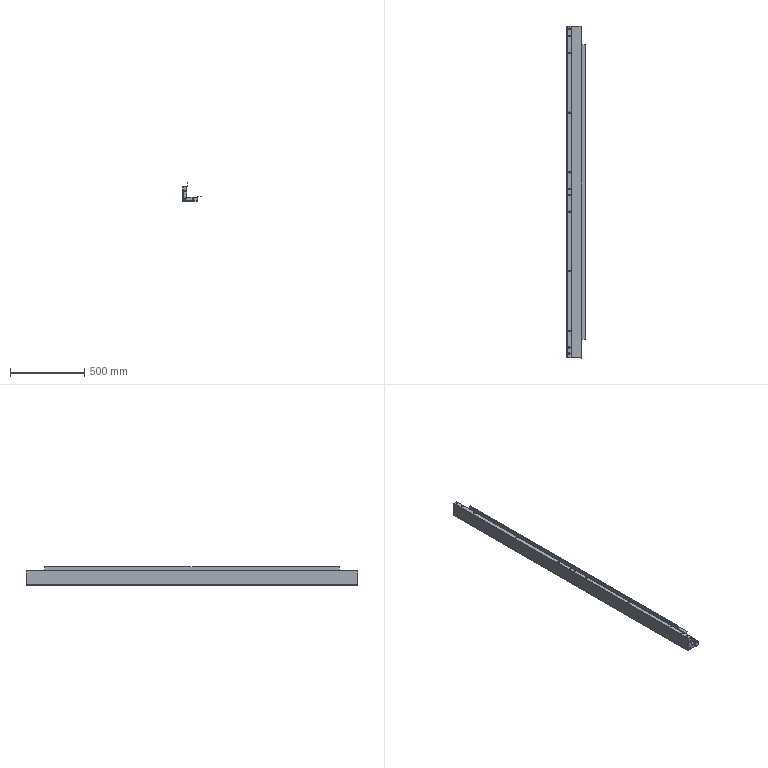Component | SolidWorks | 11LeftRearColumn-1 | 1 solid | 125 faces | volume 1330891 mm3 | cylinder 69 | plane 54 | spline 2 | commonest cylinder face diameters 10 x55 6 x7 2 x7